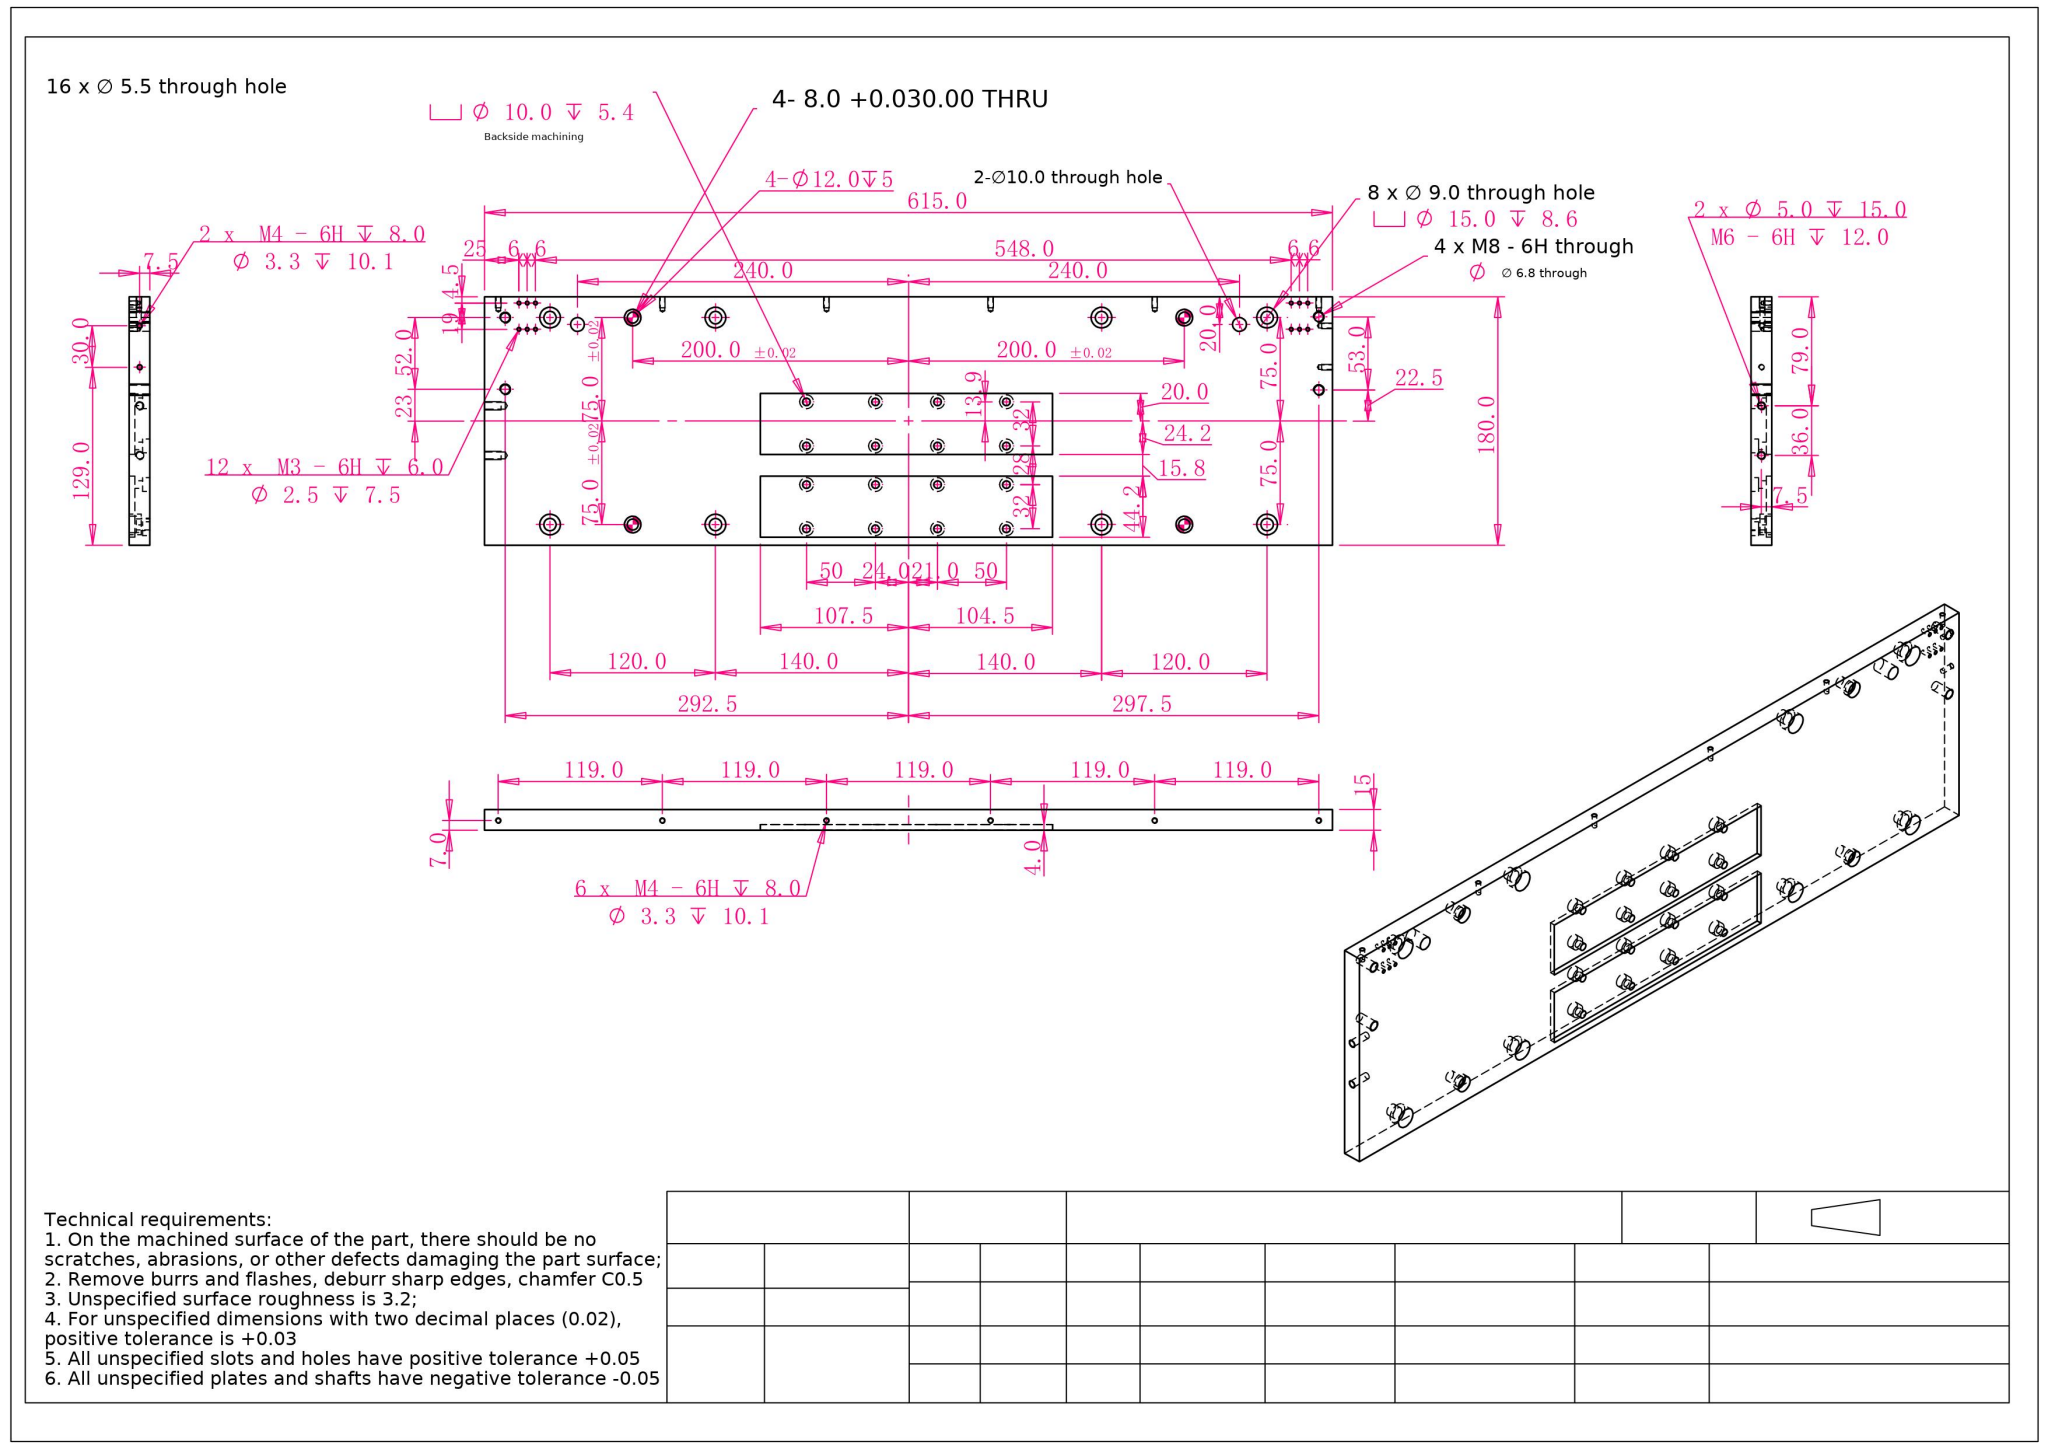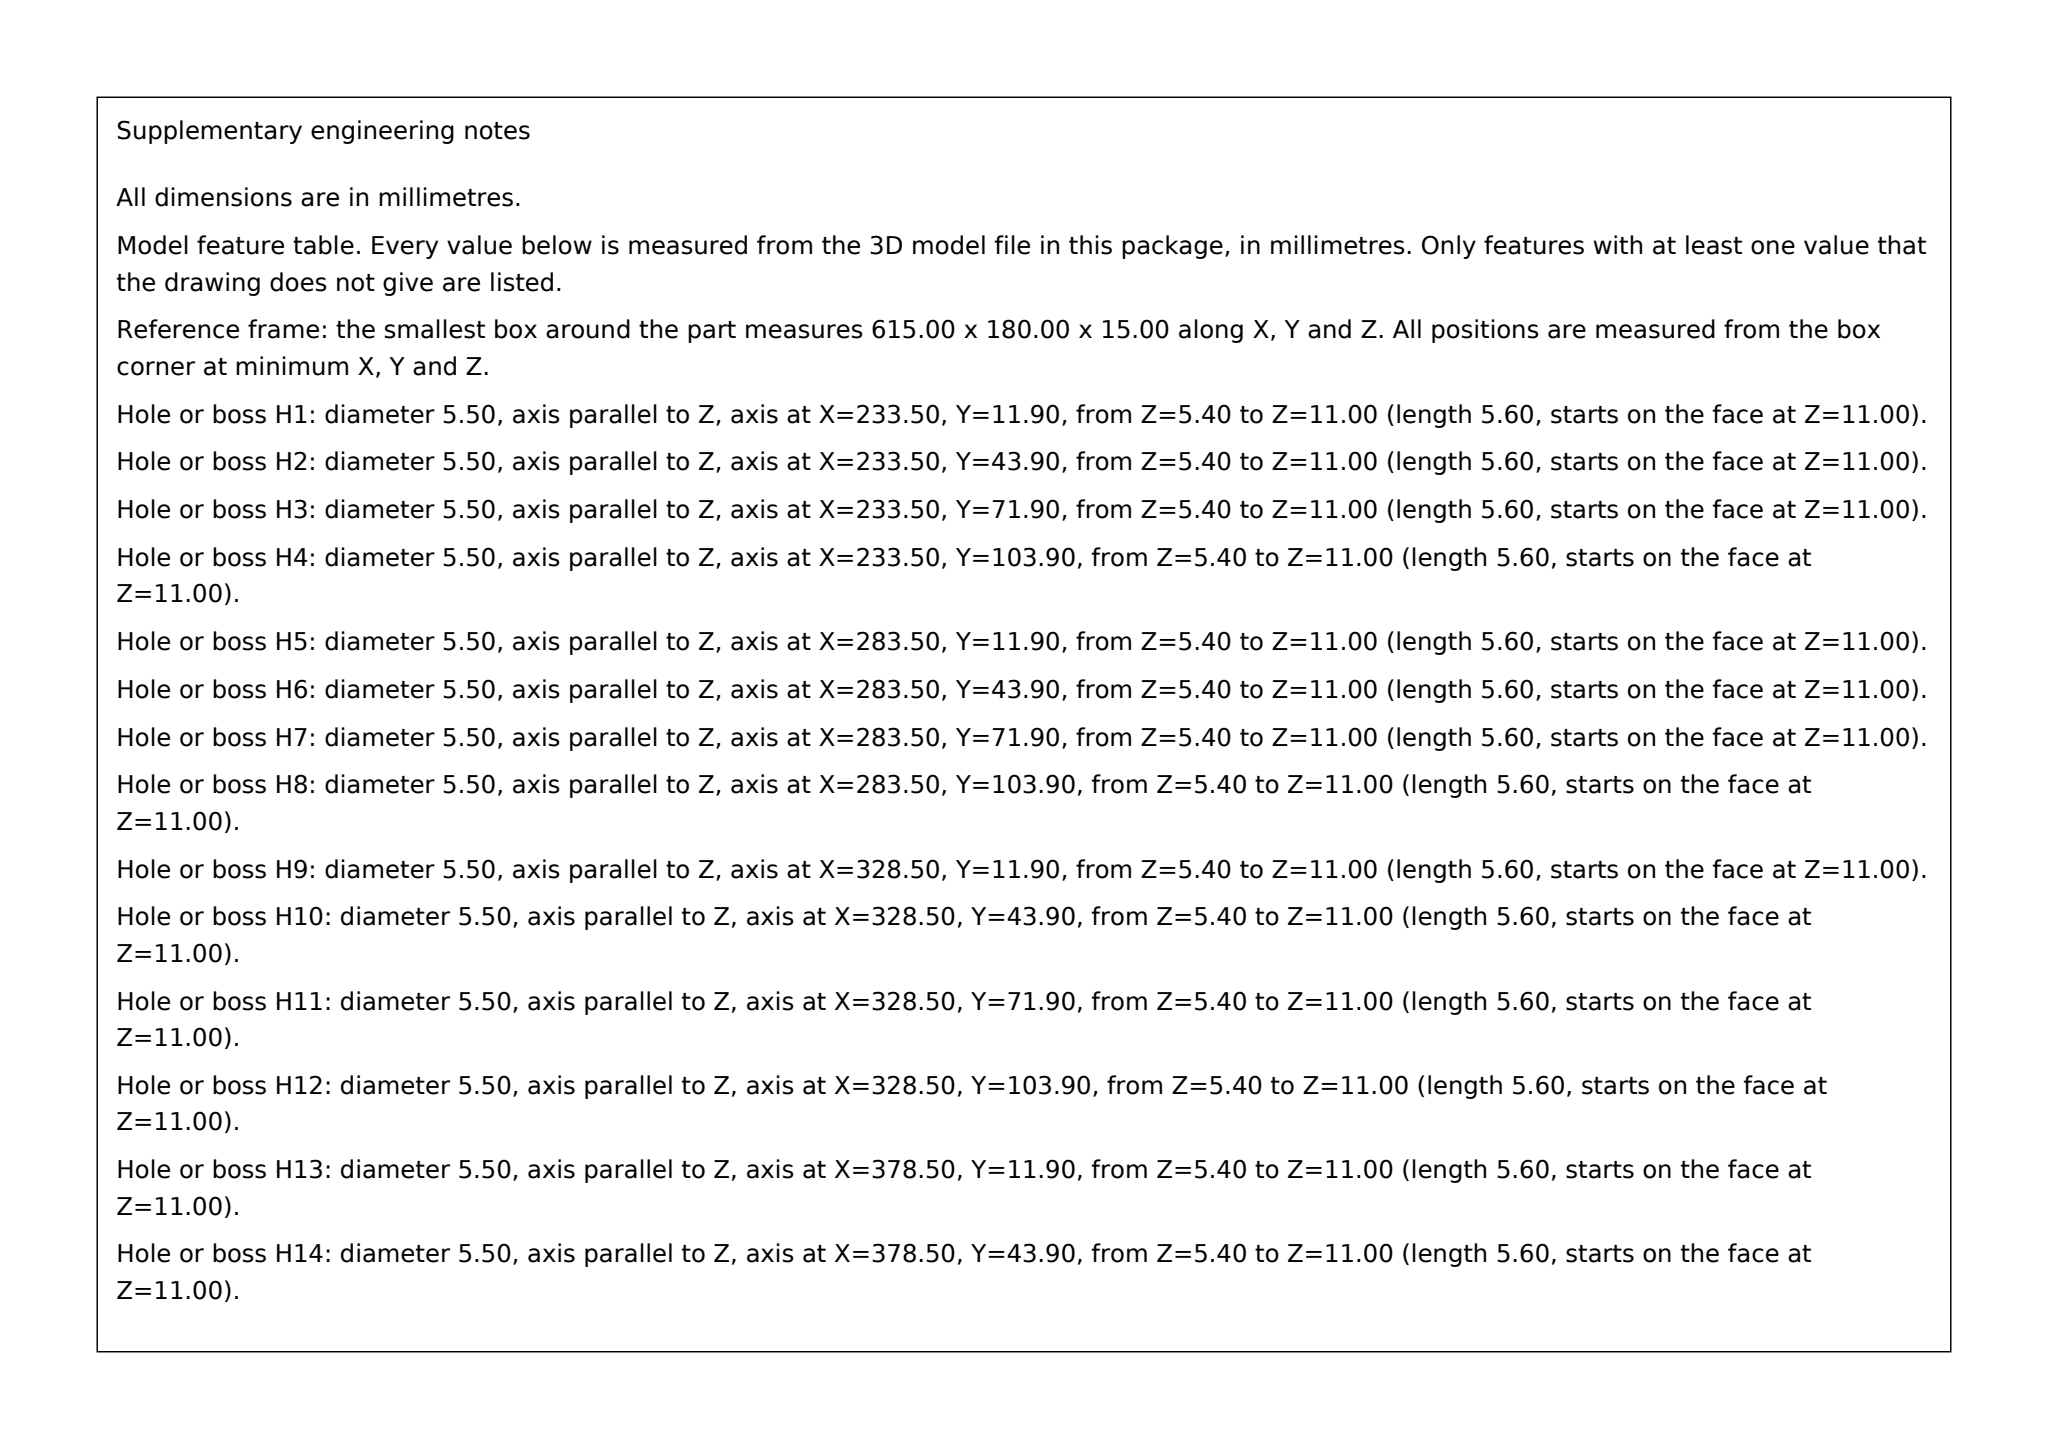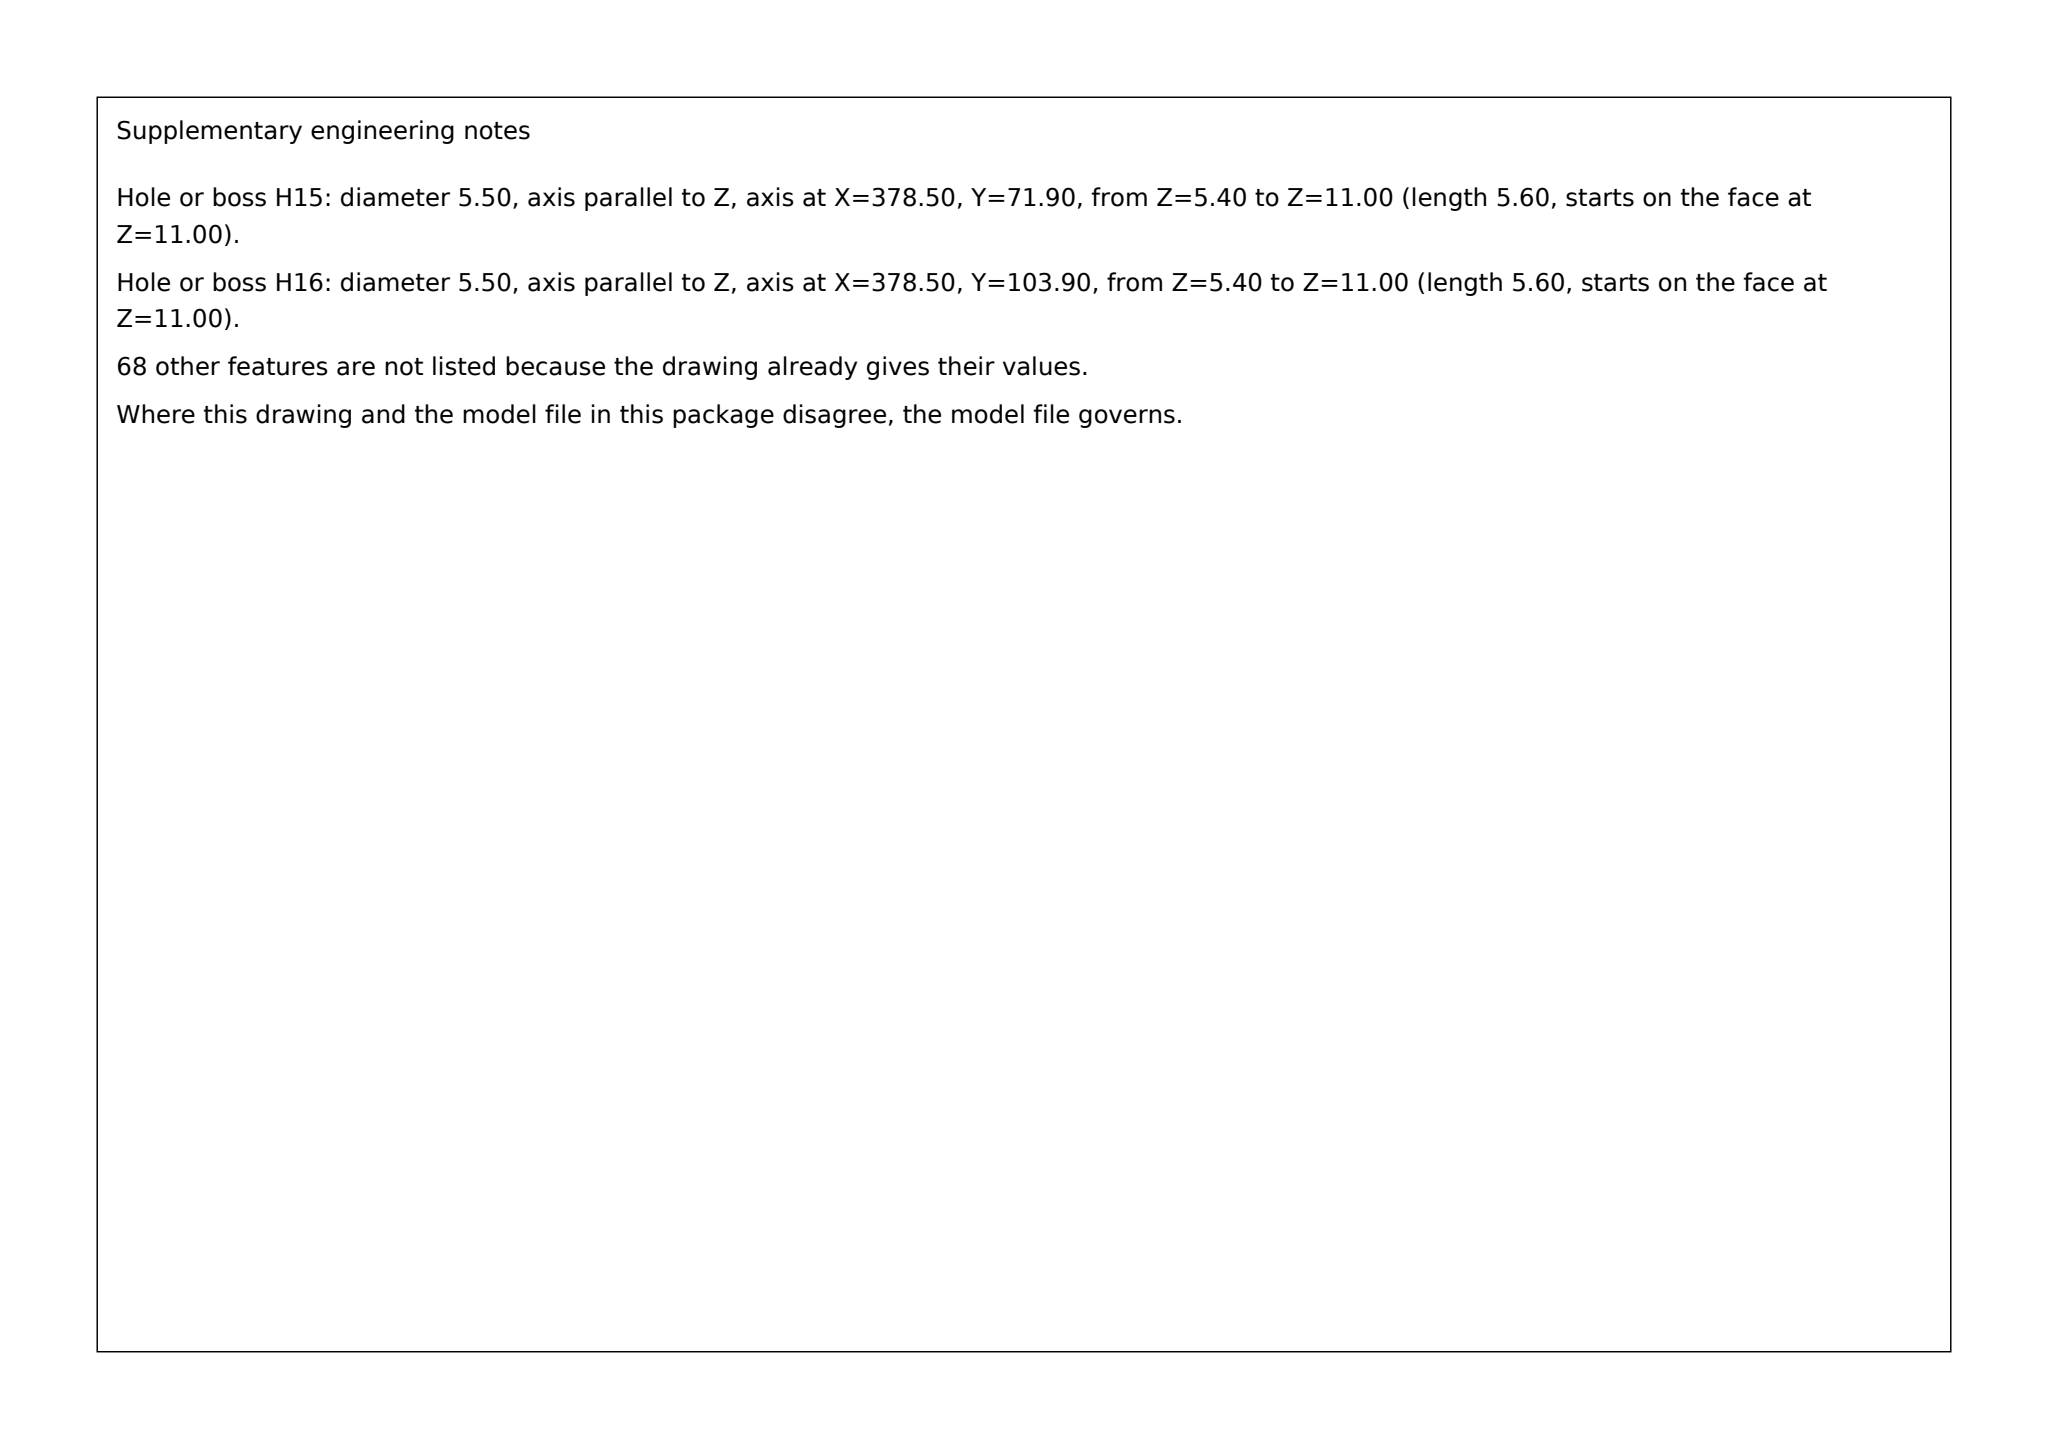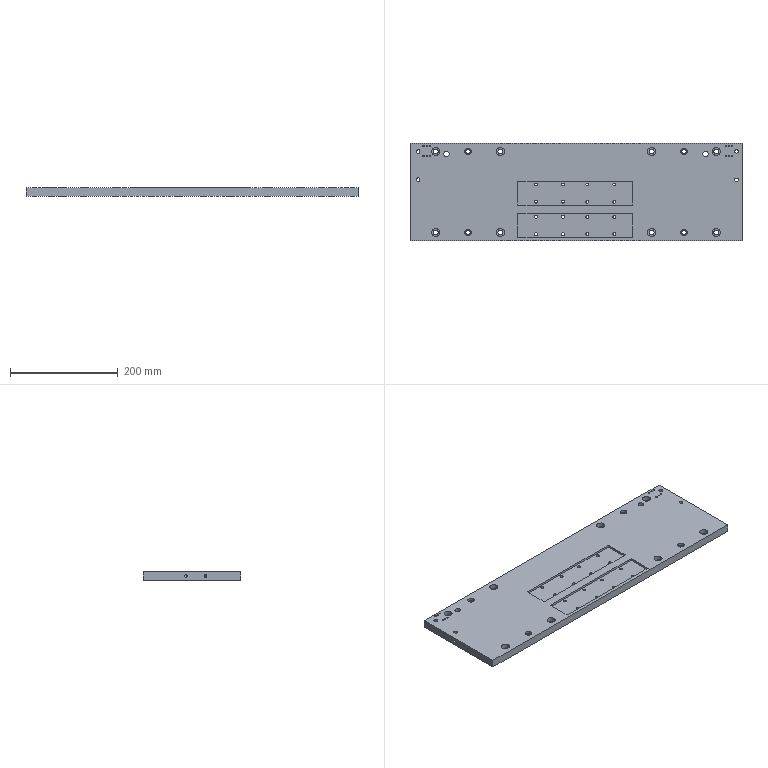Part | SolidWorks | mm | 1 solid | 256 faces | box 615 x 180 x 15 mm | volume 1550620 mm3 | cylinder 168 | cone 44 | plane 44 | commonest cylinder face diameters 10 x36 5.5 x32 2.5 x24 3.3 x16 15 x16 9 x16 12 x8 6.8 x8
build123d program:
from build123d import *

# Parameters (mm, degrees)
SKETCH1_W                                       = 615
SKETCH1_H                                       = 180
BOSS_EXTRUDE1_DEPTH                             = 15
M8_TAPPED_HOLE1_D                               = 6.8
SKETCH11_W                                      = 212
SKETCH11_H                                      = 44.2
CUT_EXTRUDE3_DEPTH                              = 4
M5_HEX_SOCKET_HEAD_CAP_SCREW_CBORE1_D           = 5.5
M5_HEX_SOCKET_HEAD_CAP_SCREW_CBORE1_CBORE_D     = 10
M5_HEX_SOCKET_HEAD_CAP_SCREW_CBORE1_CBORE_DEPTH = 5.4
M8_HEX_SOCKET_HEAD_CAP_SCREW_CBORE1_D           = 9
M8_HEX_SOCKET_HEAD_CAP_SCREW_CBORE1_CBORE_D     = 15
M8_HEX_SOCKET_HEAD_CAP_SCREW_CBORE1_CBORE_DEPTH = 8.6
M4_TAPPED_HOLE1_D                               = 3.3
M4_TAPPED_HOLE1_DEPTH                           = 10.1
M4_TAPPED_HOLE1_TIP                             = 0.9914
M3_TAPPED_HOLE2_D                               = 2.5
M3_TAPPED_HOLE2_DEPTH                           = 7.5
M3_TAPPED_HOLE2_TIP                             = 0.7511
M6_TAPPED_HOLE1_D                               = 5
M6_TAPPED_HOLE1_DEPTH                           = 15
M6_TAPPED_HOLE1_TIP                             = 1.502
M4_TAPPED_HOLE2_D                               = 3.3
M4_TAPPED_HOLE2_DEPTH                           = 10.1
M4_TAPPED_HOLE2_TIP                             = 0.9914
SKETCH34_R                                      = 4
CUT_EXTRUDE6_DEPTH                              = 321.751
SKETCH35_R                                      = 6
CUT_EXTRUDE7_DEPTH                              = 5
SKETCH36_W                                      = 14.5
SKETCH36_H                                      = 24.75
BOSS_EXTRUDE5_DEPTH                             = 15
CUT_EXTRUDE8_DEPTH                              = 321.751
CUT_EXTRUDE8_DEPTH_BACK                         = 321.751
SKETCH37_R                                      = 5


with BuildPart() as part:
    # Sketch1 → Boss-Extrude1 (new body)
    with BuildSketch(Plane.XY):
        Rectangle(SKETCH1_W, SKETCH1_H)
    extrude(amount=BOSS_EXTRUDE1_DEPTH)

    # M8 Tapped Hole1 (through all)
    with Locations(Plane.XY.offset(15)):
        with Locations((-292.5, 75), (-292.5, 23), (297.5, 75.5), (297.5, 22.5)):
            Hole(M8_TAPPED_HOLE1_D / 2)

    # Sketch11 → Cut-Extrude3 (cut)
    with BuildSketch(Plane.XY.offset(15)):
        with Locations((-1.5, -2.1)):
            Rectangle(SKETCH11_W, SKETCH11_H)
        with Locations((-1.5, -62.1)):
            Rectangle(SKETCH11_W, SKETCH11_H)
    extrude(amount=-CUT_EXTRUDE3_DEPTH, mode=Mode.SUBTRACT)

    # M5 Hex Socket Head Cap Screw CBORE1 (through all)
    with Locations(Plane(origin=(0, 0, 0), x_dir=(-1, 0, 0), z_dir=(0, 0, -1))):
        with Locations((74, -46.1), (24, -46.1), (24, -78.1), (74, -78.1), (-71, -78.1), (-21, -78.1), (-21, -46.1), (-71, -46.1), (-71, -18.1), (-21, -18.1), (-21, 13.9), (-71, 13.9), (74, 13.9), (24, 13.9), (24, -18.1), (74, -18.1)):
            CounterBoreHole(M5_HEX_SOCKET_HEAD_CAP_SCREW_CBORE1_D / 2, M5_HEX_SOCKET_HEAD_CAP_SCREW_CBORE1_CBORE_D / 2, M5_HEX_SOCKET_HEAD_CAP_SCREW_CBORE1_CBORE_DEPTH)

    # M8 Hex Socket Head Cap Screw CBORE1 (through all)
    with Locations(Plane.XY.offset(15)):
        with Locations((260, -75), (140, -75), (140, 75), (260, 75), (-260, 75), (-140, 75), (-140, -75), (-260, -75)):
            CounterBoreHole(M8_HEX_SOCKET_HEAD_CAP_SCREW_CBORE1_D / 2, M8_HEX_SOCKET_HEAD_CAP_SCREW_CBORE1_CBORE_D / 2, M8_HEX_SOCKET_HEAD_CAP_SCREW_CBORE1_CBORE_DEPTH)

    # M4 Tapped Hole1
    with Locations(Plane(origin=(0, 90, 0), x_dir=(-1, 0, 0), z_dir=(0, 1, 0))):
        with Locations((297.5, 8), (178.5, 8), (59.5, 8), (-59.5, 8), (-178.5, 8), (-297.5, 8)):
            Hole(M4_TAPPED_HOLE1_D / 2, depth=M4_TAPPED_HOLE1_DEPTH)
            with Locations((0, 0, -(M4_TAPPED_HOLE1_DEPTH + M4_TAPPED_HOLE1_TIP / 2))):  # 118° drill point
                Cone(0, M4_TAPPED_HOLE1_D / 2, M4_TAPPED_HOLE1_TIP, mode=Mode.SUBTRACT)

    # M3 Tapped Hole2
    with Locations(Plane.XY.offset(15)):
        with Locations((-282.5, 66.5), (-282.5, -66.5), (-282.5, -85.5), (-276.5, -85.5), (-276.5, -66.5), (-270.5, -66.5), (-270.5, -85.5), (277.5, -85.5), (277.5, -66.5), (283.5, -66.5), (283.5, -85.5), (289.5, -85.5), (289.5, -66.5), (289.5, 66.5), (289.5, 85.5), (283.5, 85.5), (283.5, 66.5), (277.5, 66.5), (277.5, 85.5), (-270.5, 85.5), (-270.5, 66.5), (-276.5, 66.5), (-276.5, 85.5), (-282.5, 85.5)):
            Hole(M3_TAPPED_HOLE2_D / 2, depth=M3_TAPPED_HOLE2_DEPTH)
            with Locations((0, 0, -(M3_TAPPED_HOLE2_DEPTH + M3_TAPPED_HOLE2_TIP / 2))):  # 118° drill point
                Cone(0, M3_TAPPED_HOLE2_D / 2, M3_TAPPED_HOLE2_TIP, mode=Mode.SUBTRACT)

    # M6 Tapped Hole1
    with Locations(Plane.ZY.offset(307.5)):
        with Locations((7.5, 11), (7.5, -25)):
            Hole(M6_TAPPED_HOLE1_D / 2, depth=M6_TAPPED_HOLE1_DEPTH)
            with Locations((0, 0, -(M6_TAPPED_HOLE1_DEPTH + M6_TAPPED_HOLE1_TIP / 2))):  # 118° drill point
                Cone(0, M6_TAPPED_HOLE1_D / 2, M6_TAPPED_HOLE1_TIP, mode=Mode.SUBTRACT)

    # M4 Tapped Hole2
    with Locations(Plane(origin=(307.5, 0, 0), x_dir=(0, 0, -1), z_dir=(1, 0, 0))):
        with Locations((-7.5, 39), (-7.5, 69)):
            Hole(M4_TAPPED_HOLE2_D / 2, depth=M4_TAPPED_HOLE2_DEPTH)
            with Locations((0, 0, -(M4_TAPPED_HOLE2_DEPTH + M4_TAPPED_HOLE2_TIP / 2))):  # 118° drill point
                Cone(0, M4_TAPPED_HOLE2_D / 2, M4_TAPPED_HOLE2_TIP, mode=Mode.SUBTRACT)

    # Sketch34 → Cut-Extrude6 (cut, through all)
    with BuildSketch(Plane.XY.offset(15)):
        with Locations((-200, 75)):
            Circle(SKETCH34_R)
        with Locations(Location((200, 75, 0), (0, 0, 180))):
            Circle(SKETCH34_R)
        with Locations((200, -75)):
            Circle(SKETCH34_R)
        with Locations(Location((-200, -75, 0), (0, 0, 180))):
            Circle(SKETCH34_R)
    extrude(amount=-CUT_EXTRUDE6_DEPTH, mode=Mode.SUBTRACT)

    # Sketch35 → Cut-Extrude7 (cut)
    with BuildSketch(Plane.XY.offset(15)):
        with Locations((-200, 75)):
            Circle(SKETCH35_R)
        with Locations((-200, -75)):
            Circle(SKETCH35_R)
        with Locations((200, 75)):
            Circle(SKETCH35_R)
        with Locations((200, -75)):
            Circle(SKETCH35_R)
    extrude(amount=-CUT_EXTRUDE7_DEPTH, mode=Mode.SUBTRACT)

    # Sketch36 → Boss-Extrude5 (add)
    with BuildSketch(Plane.XY.offset(15)):
        with Locations((283.5, -77.625)):
            Rectangle(SKETCH36_W, SKETCH36_H)
        with Locations((-276.5, -77.625)):
            Rectangle(SKETCH36_W, SKETCH36_H)
    extrude(amount=-BOSS_EXTRUDE5_DEPTH)

    # Sketch37 → Cut-Extrude8 (cut, two sides: drawn at the far end of the back side and taken through both)
    with BuildSketch(Plane.XY.offset(15).offset(-CUT_EXTRUDE8_DEPTH_BACK)):
        with Locations((240, 70)):
            Circle(SKETCH37_R)
        with Locations(Location((-240, 70, 0), (0, 0, 180))):
            Circle(SKETCH37_R)
    extrude(amount=CUT_EXTRUDE8_DEPTH + CUT_EXTRUDE8_DEPTH_BACK, mode=Mode.SUBTRACT)


solid = part.part